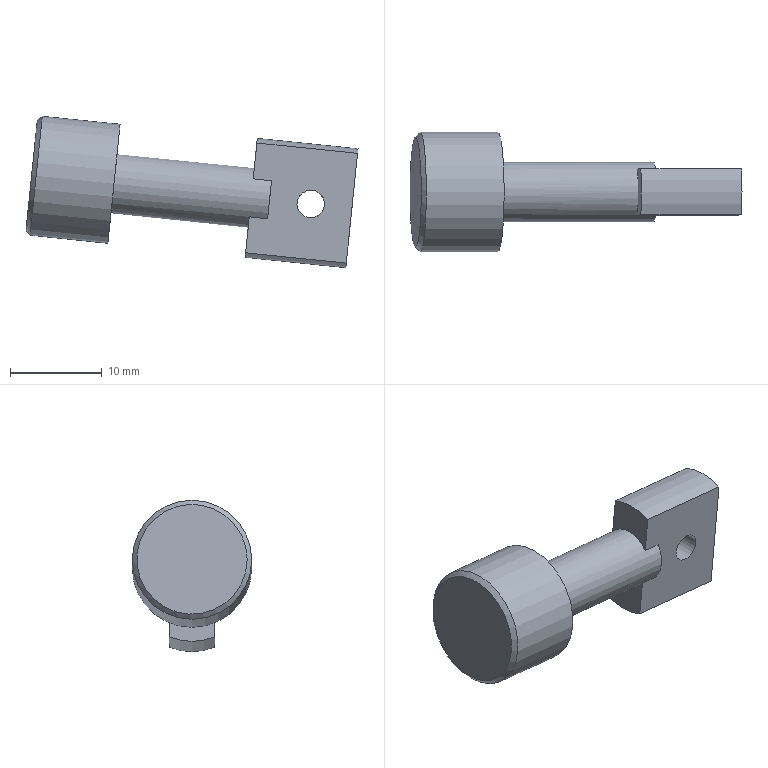Component | NX | PISTON | 1 solid | 15 faces | box 36.09 x 13 x 16.46 mm | volume 2357 mm3 | plane 9 | cylinder 5 | cone 1 | commonest cylinder face diameters 13 x3 6.5 x1 3 x1
STEP:
#1=CARTESIAN_POINT('',(0.,0.,0.));
#2=DIRECTION('',(0.,0.,1.));
#3=DIRECTION('',(1.,0.,0.));
#4=AXIS2_PLACEMENT_3D('',#1,#2,#3);
#5=CARTESIAN_POINT('',(20.798,-27.5,35.026));
#6=VERTEX_POINT('',#5);
#7=CARTESIAN_POINT('',(20.373,-27.5,30.894));
#8=VERTEX_POINT('',#7);
#9=CARTESIAN_POINT('',(20.586,-27.5,32.96));
#10=DIRECTION('',(-0.1022,0.,-0.9948));
#11=VECTOR('',#10,1.);
#12=LINE('',#9,#11);
#13=CARTESIAN_POINT('',(20.586,-30.,32.96));
#14=DIRECTION('',(0.9948,0.,-0.1022));
#15=DIRECTION('',(0.,1.,0.));
#16=AXIS2_PLACEMENT_3D('',#13,#14,#15);
#17=PLANE('',#16);
#18=CARTESIAN_POINT('',(2.5,0.));
#19=DIRECTION('',(0.,-1.));
#20=VECTOR('',#19,1.);
#21=LINE('',#18,#20);
#22=(GEOMETRIC_REPRESENTATION_CONTEXT(2)PARAMETRIC_REPRESENTATION_CONTEXT()REPRESENTATION_CONTEXT('',''));
#23=DEFINITIONAL_REPRESENTATION('',(#21),#22);
#24=PCURVE('',#17,#23);
#25=CARTESIAN_POINT('',(30.152,-27.5,38.009));
#26=DIRECTION('',(0.,1.,0.));
#27=DIRECTION('',(-0.9948,0.,0.1022));
#28=AXIS2_PLACEMENT_3D('',#25,#26,#27);
#29=PLANE('',#28);
#30=CARTESIAN_POINT('',(9.,-6.));
#31=DIRECTION('',(-0.,-1.));
#32=VECTOR('',#31,1.);
#33=LINE('',#30,#32);
#34=(GEOMETRIC_REPRESENTATION_CONTEXT(2)PARAMETRIC_REPRESENTATION_CONTEXT()REPRESENTATION_CONTEXT('',''));
#35=DEFINITIONAL_REPRESENTATION('',(#33),#34);
#36=PCURVE('',#29,#35);
#37=SURFACE_CURVE('',#12,(#24,#36),.PCURVE_S1.);
#38=EDGE_CURVE('',#6,#8,#37,.T.);
#39=ORIENTED_EDGE('',*,*,#38,.T.);
#40=CARTESIAN_POINT('',(20.586,-26.75,32.96));
#41=VERTEX_POINT('',#40);
#42=CARTESIAN_POINT('',(20.586,-30.,32.96));
#43=DIRECTION('',(0.9948,0.,-0.1022));
#44=DIRECTION('',(0.,1.,0.));
#45=AXIS2_PLACEMENT_3D('',#42,#43,#44);
#46=CIRCLE('',#45,3.25);
#47=CARTESIAN_POINT('',(0.,0.));
#48=DIRECTION('',(1.,0.));
#49=AXIS2_PLACEMENT_2D('',#47,#48);
#50=CIRCLE('',#49,3.25);
#51=(GEOMETRIC_REPRESENTATION_CONTEXT(2)PARAMETRIC_REPRESENTATION_CONTEXT()REPRESENTATION_CONTEXT('',''));
#52=DEFINITIONAL_REPRESENTATION('',(#50),#51);
#53=PCURVE('',#17,#52);
#54=CARTESIAN_POINT('',(3.675,-30.,34.698));
#55=DIRECTION('',(0.9948,0.,-0.1022));
#56=DIRECTION('',(0.,1.,0.));
#57=AXIS2_PLACEMENT_3D('',#54,#55,#56);
#58=CYLINDRICAL_SURFACE('',#57,3.25);
#59=CARTESIAN_POINT('',(0.,17.));
#60=DIRECTION('',(1.,0.));
#61=VECTOR('',#60,1.);
#62=LINE('',#59,#61);
#63=(GEOMETRIC_REPRESENTATION_CONTEXT(2)PARAMETRIC_REPRESENTATION_CONTEXT()REPRESENTATION_CONTEXT('',''));
#64=DEFINITIONAL_REPRESENTATION('',(#62),#63);
#65=PCURVE('',#58,#64);
#66=SURFACE_CURVE('',#46,(#53,#65),.PCURVE_S1.);
#67=EDGE_CURVE('',#8,#41,#66,.T.);
#68=ORIENTED_EDGE('',*,*,#67,.T.);
#69=CARTESIAN_POINT('',(20.586,-30.,32.96));
#70=DIRECTION('',(0.9948,0.,-0.1022));
#71=DIRECTION('',(0.,1.,0.));
#72=AXIS2_PLACEMENT_3D('',#69,#70,#71);
#73=CIRCLE('',#72,3.25);
#74=CARTESIAN_POINT('',(0.,0.));
#75=DIRECTION('',(1.,0.));
#76=AXIS2_PLACEMENT_2D('',#74,#75);
#77=CIRCLE('',#76,3.25);
#78=(GEOMETRIC_REPRESENTATION_CONTEXT(2)PARAMETRIC_REPRESENTATION_CONTEXT()REPRESENTATION_CONTEXT('',''));
#79=DEFINITIONAL_REPRESENTATION('',(#77),#78);
#80=PCURVE('',#17,#79);
#81=CARTESIAN_POINT('',(-6.283,17.));
#82=DIRECTION('',(1.,0.));
#83=VECTOR('',#82,1.);
#84=LINE('',#81,#83);
#85=(GEOMETRIC_REPRESENTATION_CONTEXT(2)PARAMETRIC_REPRESENTATION_CONTEXT()REPRESENTATION_CONTEXT('',''));
#86=DEFINITIONAL_REPRESENTATION('',(#84),#85);
#87=PCURVE('',#58,#86);
#88=SURFACE_CURVE('',#73,(#80,#87),.PCURVE_S1.);
#89=EDGE_CURVE('',#41,#6,#88,.T.);
#90=ORIENTED_EDGE('',*,*,#89,.T.);
#91=EDGE_LOOP('',(#39,#68,#90));
#92=FACE_BOUND('',#91,.T.);
#93=ADVANCED_FACE('',(#92),#17,.T.);
#94=CARTESIAN_POINT('',(3.675,-26.75,34.698));
#95=VERTEX_POINT('',#94);
#96=CARTESIAN_POINT('',(3.675,-30.,34.698));
#97=DIRECTION('',(0.9948,0.,-0.1022));
#98=DIRECTION('',(0.,1.,0.));
#99=AXIS2_PLACEMENT_3D('',#96,#97,#98);
#100=CIRCLE('',#99,3.25);
#101=CARTESIAN_POINT('',(3.675,-30.,34.698));
#102=DIRECTION('',(0.9948,0.,-0.1022));
#103=DIRECTION('',(0.,1.,0.));
#104=AXIS2_PLACEMENT_3D('',#101,#102,#103);
#105=PLANE('',#104);
#106=CARTESIAN_POINT('',(0.,0.));
#107=DIRECTION('',(1.,0.));
#108=AXIS2_PLACEMENT_2D('',#106,#107);
#109=CIRCLE('',#108,3.25);
#110=(GEOMETRIC_REPRESENTATION_CONTEXT(2)PARAMETRIC_REPRESENTATION_CONTEXT()REPRESENTATION_CONTEXT('',''));
#111=DEFINITIONAL_REPRESENTATION('',(#109),#110);
#112=PCURVE('',#105,#111);
#113=CARTESIAN_POINT('',(0.,0.));
#114=DIRECTION('',(1.,0.));
#115=VECTOR('',#114,1.);
#116=LINE('',#113,#115);
#117=(GEOMETRIC_REPRESENTATION_CONTEXT(2)PARAMETRIC_REPRESENTATION_CONTEXT()REPRESENTATION_CONTEXT('',''));
#118=DEFINITIONAL_REPRESENTATION('',(#116),#117);
#119=PCURVE('',#58,#118);
#120=SURFACE_CURVE('',#100,(#112,#119),.PCURVE_S1.);
#121=EDGE_CURVE('',#95,#95,#120,.T.);
#122=ORIENTED_EDGE('',*,*,#121,.F.);
#123=EDGE_LOOP('',(#122));
#124=FACE_BOUND('',#123,.T.);
#125=CARTESIAN_POINT('',(3.675,-23.5,34.698));
#126=VERTEX_POINT('',#125);
#127=CARTESIAN_POINT('',(3.675,-30.,34.698));
#128=DIRECTION('',(-0.9948,0.,0.1022));
#129=DIRECTION('',(0.,1.,0.));
#130=AXIS2_PLACEMENT_3D('',#127,#128,#129);
#131=CIRCLE('',#130,6.5);
#132=CARTESIAN_POINT('',(6.5,0.));
#133=CARTESIAN_POINT('',(6.5,-11.258));
#134=CARTESIAN_POINT('',(-3.25,-5.629));
#135=CARTESIAN_POINT('',(-13.,-0.));
#136=CARTESIAN_POINT('',(-3.25,5.629));
#137=CARTESIAN_POINT('',(6.5,11.258));
#138=CARTESIAN_POINT('',(6.5,0.));
#139=(BOUNDED_CURVE()B_SPLINE_CURVE(2,(#132,#133,#134,#135,#136,#137,#138),.UNSPECIFIED.,.T.,.F.)B_SPLINE_CURVE_WITH_KNOTS((1,2,2,2,2,1),(-2.094,0.,2.094,4.189,6.283,8.378),.UNSPECIFIED.)CURVE()GEOMETRIC_REPRESENTATION_ITEM()RATIONAL_B_SPLINE_CURVE((1.,0.5,1.,0.5,1.,0.5,1.))REPRESENTATION_ITEM(''));
#140=(GEOMETRIC_REPRESENTATION_CONTEXT(2)PARAMETRIC_REPRESENTATION_CONTEXT()REPRESENTATION_CONTEXT('',''));
#141=DEFINITIONAL_REPRESENTATION('',(#139),#140);
#142=PCURVE('',#105,#141);
#143=CARTESIAN_POINT('',(-5.278,-30.,35.618));
#144=DIRECTION('',(0.9948,0.,-0.1022));
#145=DIRECTION('',(0.,1.,0.));
#146=AXIS2_PLACEMENT_3D('',#143,#144,#145);
#147=CYLINDRICAL_SURFACE('',#146,6.5);
#148=CARTESIAN_POINT('',(6.283,9.));
#149=DIRECTION('',(-1.,0.));
#150=VECTOR('',#149,1.);
#151=LINE('',#148,#150);
#152=(GEOMETRIC_REPRESENTATION_CONTEXT(2)PARAMETRIC_REPRESENTATION_CONTEXT()REPRESENTATION_CONTEXT('',''));
#153=DEFINITIONAL_REPRESENTATION('',(#151),#152);
#154=PCURVE('',#147,#153);
#155=SURFACE_CURVE('',#131,(#142,#154),.PCURVE_S1.);
#156=EDGE_CURVE('',#126,#126,#155,.T.);
#157=ORIENTED_EDGE('',*,*,#156,.F.);
#158=EDGE_LOOP('',(#157));
#159=FACE_BOUND('',#158,.T.);
#160=ADVANCED_FACE('',(#124,#159),#105,.T.);
#161=CARTESIAN_POINT('',(-5.278,-36.,35.618));
#162=VERTEX_POINT('',#161);
#163=CARTESIAN_POINT('',(-5.278,-30.,35.618));
#164=DIRECTION('',(-0.9948,0.,0.1022));
#165=DIRECTION('',(0.,-1.,0.));
#166=AXIS2_PLACEMENT_3D('',#163,#164,#165);
#167=CIRCLE('',#166,6.);
#168=CARTESIAN_POINT('',(-5.278,-30.,35.618));
#169=DIRECTION('',(-0.9948,0.,0.1022));
#170=DIRECTION('',(0.,-1.,0.));
#171=AXIS2_PLACEMENT_3D('',#168,#169,#170);
#172=PLANE('',#171);
#173=CARTESIAN_POINT('',(0.,0.));
#174=DIRECTION('',(1.,0.));
#175=AXIS2_PLACEMENT_2D('',#173,#174);
#176=CIRCLE('',#175,6.);
#177=(GEOMETRIC_REPRESENTATION_CONTEXT(2)PARAMETRIC_REPRESENTATION_CONTEXT()REPRESENTATION_CONTEXT('',''));
#178=DEFINITIONAL_REPRESENTATION('',(#176),#177);
#179=PCURVE('',#172,#178);
#180=CARTESIAN_POINT('',(-4.781,-30.,35.566));
#181=DIRECTION('',(0.9948,0.,-0.1022));
#182=DIRECTION('',(0.,1.,0.));
#183=AXIS2_PLACEMENT_3D('',#180,#181,#182);
#184=CONICAL_SURFACE('',#183,6.5,0.7854);
#185=CARTESIAN_POINT('',(9.425,-0.5));
#186=DIRECTION('',(-1.,0.));
#187=VECTOR('',#186,1.);
#188=LINE('',#185,#187);
#189=(GEOMETRIC_REPRESENTATION_CONTEXT(2)PARAMETRIC_REPRESENTATION_CONTEXT()REPRESENTATION_CONTEXT('',''));
#190=DEFINITIONAL_REPRESENTATION('',(#188),#189);
#191=PCURVE('',#184,#190);
#192=SURFACE_CURVE('',#167,(#179,#191),.PCURVE_S1.);
#193=EDGE_CURVE('',#162,#162,#192,.T.);
#194=ORIENTED_EDGE('',*,*,#193,.T.);
#195=EDGE_LOOP('',(#194));
#196=FACE_BOUND('',#195,.T.);
#197=ADVANCED_FACE('',(#196),#172,.T.);
#198=CARTESIAN_POINT('',(-4.781,-36.5,35.566));
#199=VERTEX_POINT('',#198);
#200=CARTESIAN_POINT('',(-4.781,-23.5,35.566));
#201=VERTEX_POINT('',#200);
#202=CARTESIAN_POINT('',(-4.781,-30.,35.566));
#203=DIRECTION('',(0.9948,0.,-0.1022));
#204=DIRECTION('',(0.,-1.,0.));
#205=AXIS2_PLACEMENT_3D('',#202,#203,#204);
#206=CIRCLE('',#205,6.5);
#207=CARTESIAN_POINT('',(3.142,0.5));
#208=DIRECTION('',(1.,0.));
#209=VECTOR('',#208,1.);
#210=LINE('',#207,#209);
#211=(GEOMETRIC_REPRESENTATION_CONTEXT(2)PARAMETRIC_REPRESENTATION_CONTEXT()REPRESENTATION_CONTEXT('',''));
#212=DEFINITIONAL_REPRESENTATION('',(#210),#211);
#213=PCURVE('',#147,#212);
#214=CARTESIAN_POINT('',(3.142,0.));
#215=DIRECTION('',(1.,0.));
#216=VECTOR('',#215,1.);
#217=LINE('',#214,#216);
#218=(GEOMETRIC_REPRESENTATION_CONTEXT(2)PARAMETRIC_REPRESENTATION_CONTEXT()REPRESENTATION_CONTEXT('',''));
#219=DEFINITIONAL_REPRESENTATION('',(#217),#218);
#220=PCURVE('',#184,#219);
#221=SURFACE_CURVE('',#206,(#213,#220),.PCURVE_S1.);
#222=EDGE_CURVE('',#199,#201,#221,.T.);
#223=ORIENTED_EDGE('',*,*,#222,.T.);
#224=CARTESIAN_POINT('',(-4.781,-23.5,35.566));
#225=CARTESIAN_POINT('',(3.675,-23.5,34.698));
#226=B_SPLINE_CURVE_WITH_KNOTS('',1,(#224,#225),.UNSPECIFIED.,.F.,.F.,(2,2),(0.5,9.),.PIECEWISE_BEZIER_KNOTS.);
#227=CARTESIAN_POINT('',(6.283,0.));
#228=DIRECTION('',(0.,1.));
#229=VECTOR('',#228,1.);
#230=LINE('',#227,#229);
#231=(GEOMETRIC_REPRESENTATION_CONTEXT(2)PARAMETRIC_REPRESENTATION_CONTEXT()REPRESENTATION_CONTEXT('',''));
#232=DEFINITIONAL_REPRESENTATION('',(#230),#231);
#233=PCURVE('',#147,#232);
#234=CARTESIAN_POINT('',(0.,0.));
#235=DIRECTION('',(0.,1.));
#236=VECTOR('',#235,1.);
#237=LINE('',#234,#236);
#238=(GEOMETRIC_REPRESENTATION_CONTEXT(2)PARAMETRIC_REPRESENTATION_CONTEXT()REPRESENTATION_CONTEXT('',''));
#239=DEFINITIONAL_REPRESENTATION('',(#237),#238);
#240=PCURVE('',#147,#239);
#241=SEAM_CURVE('',#226,(#233,#240),.PCURVE_S1.);
#242=EDGE_CURVE('',#201,#126,#241,.T.);
#243=ORIENTED_EDGE('',*,*,#242,.T.);
#244=ORIENTED_EDGE('',*,*,#156,.T.);
#245=ORIENTED_EDGE('',*,*,#242,.F.);
#246=CARTESIAN_POINT('',(-4.781,-30.,35.566));
#247=DIRECTION('',(0.9948,0.,-0.1022));
#248=DIRECTION('',(0.,-1.,0.));
#249=AXIS2_PLACEMENT_3D('',#246,#247,#248);
#250=CIRCLE('',#249,6.5);
#251=CARTESIAN_POINT('',(-3.142,0.5));
#252=DIRECTION('',(1.,0.));
#253=VECTOR('',#252,1.);
#254=LINE('',#251,#253);
#255=(GEOMETRIC_REPRESENTATION_CONTEXT(2)PARAMETRIC_REPRESENTATION_CONTEXT()REPRESENTATION_CONTEXT('',''));
#256=DEFINITIONAL_REPRESENTATION('',(#254),#255);
#257=PCURVE('',#147,#256);
#258=CARTESIAN_POINT('',(3.142,0.));
#259=DIRECTION('',(1.,0.));
#260=VECTOR('',#259,1.);
#261=LINE('',#258,#260);
#262=(GEOMETRIC_REPRESENTATION_CONTEXT(2)PARAMETRIC_REPRESENTATION_CONTEXT()REPRESENTATION_CONTEXT('',''));
#263=DEFINITIONAL_REPRESENTATION('',(#261),#262);
#264=PCURVE('',#184,#263);
#265=SURFACE_CURVE('',#250,(#257,#264),.PCURVE_S1.);
#266=EDGE_CURVE('',#201,#199,#265,.T.);
#267=ORIENTED_EDGE('',*,*,#266,.T.);
#268=EDGE_LOOP('',(#223,#243,#244,#245,#267));
#269=FACE_BOUND('',#268,.T.);
#270=ADVANCED_FACE('',(#269),#147,.T.);
#271=CARTESIAN_POINT('',(20.373,-32.5,30.894));
#272=VERTEX_POINT('',#271);
#273=CARTESIAN_POINT('',(20.798,-32.5,35.026));
#274=VERTEX_POINT('',#273);
#275=CARTESIAN_POINT('',(20.586,-32.5,32.96));
#276=DIRECTION('',(0.1022,0.,0.9948));
#277=VECTOR('',#276,1.);
#278=LINE('',#275,#277);
#279=CARTESIAN_POINT('',(20.586,-30.,32.96));
#280=DIRECTION('',(0.9948,0.,-0.1022));
#281=DIRECTION('',(0.,1.,0.));
#282=AXIS2_PLACEMENT_3D('',#279,#280,#281);
#283=PLANE('',#282);
#284=CARTESIAN_POINT('',(-2.5,0.));
#285=DIRECTION('',(0.,1.));
#286=VECTOR('',#285,1.);
#287=LINE('',#284,#286);
#288=(GEOMETRIC_REPRESENTATION_CONTEXT(2)PARAMETRIC_REPRESENTATION_CONTEXT()REPRESENTATION_CONTEXT('',''));
#289=DEFINITIONAL_REPRESENTATION('',(#287),#288);
#290=PCURVE('',#283,#289);
#291=CARTESIAN_POINT('',(28.925,-32.5,26.071));
#292=DIRECTION('',(0.,-1.,0.));
#293=DIRECTION('',(0.9948,0.,-0.1022));
#294=AXIS2_PLACEMENT_3D('',#291,#292,#293);
#295=PLANE('',#294);
#296=CARTESIAN_POINT('',(-9.,6.));
#297=DIRECTION('',(-0.,1.));
#298=VECTOR('',#297,1.);
#299=LINE('',#296,#298);
#300=(GEOMETRIC_REPRESENTATION_CONTEXT(2)PARAMETRIC_REPRESENTATION_CONTEXT()REPRESENTATION_CONTEXT('',''));
#301=DEFINITIONAL_REPRESENTATION('',(#299),#300);
#302=PCURVE('',#295,#301);
#303=SURFACE_CURVE('',#278,(#290,#302),.PCURVE_S1.);
#304=EDGE_CURVE('',#272,#274,#303,.T.);
#305=ORIENTED_EDGE('',*,*,#304,.T.);
#306=CARTESIAN_POINT('',(20.586,-30.,32.96));
#307=DIRECTION('',(0.9948,0.,-0.1022));
#308=DIRECTION('',(0.,1.,0.));
#309=AXIS2_PLACEMENT_3D('',#306,#307,#308);
#310=CIRCLE('',#309,3.25);
#311=CARTESIAN_POINT('',(0.,0.));
#312=DIRECTION('',(1.,0.));
#313=AXIS2_PLACEMENT_2D('',#311,#312);
#314=CIRCLE('',#313,3.25);
#315=(GEOMETRIC_REPRESENTATION_CONTEXT(2)PARAMETRIC_REPRESENTATION_CONTEXT()REPRESENTATION_CONTEXT('',''));
#316=DEFINITIONAL_REPRESENTATION('',(#314),#315);
#317=PCURVE('',#283,#316);
#318=CARTESIAN_POINT('',(-0.,17.));
#319=DIRECTION('',(1.,-0.));
#320=VECTOR('',#319,1.);
#321=LINE('',#318,#320);
#322=(GEOMETRIC_REPRESENTATION_CONTEXT(2)PARAMETRIC_REPRESENTATION_CONTEXT()REPRESENTATION_CONTEXT('',''));
#323=DEFINITIONAL_REPRESENTATION('',(#321),#322);
#324=PCURVE('',#58,#323);
#325=SURFACE_CURVE('',#310,(#317,#324),.PCURVE_S1.);
#326=EDGE_CURVE('',#274,#272,#325,.T.);
#327=ORIENTED_EDGE('',*,*,#326,.T.);
#328=EDGE_LOOP('',(#305,#327));
#329=FACE_BOUND('',#328,.T.);
#330=ADVANCED_FACE('',(#329),#283,.T.);
#331=CARTESIAN_POINT('',(18.384,-27.5,31.099));
#332=VERTEX_POINT('',#331);
#333=CARTESIAN_POINT('',(3.463,-27.5,32.632));
#334=DIRECTION('',(0.9948,0.,-0.1022));
#335=VECTOR('',#334,1.);
#336=LINE('',#333,#335);
#337=CARTESIAN_POINT('',(5.59,0.));
#338=DIRECTION('',(0.,1.));
#339=VECTOR('',#338,1.);
#340=LINE('',#337,#339);
#341=(GEOMETRIC_REPRESENTATION_CONTEXT(2)PARAMETRIC_REPRESENTATION_CONTEXT()REPRESENTATION_CONTEXT('',''));
#342=DEFINITIONAL_REPRESENTATION('',(#340),#341);
#343=PCURVE('',#58,#342);
#344=CARTESIAN_POINT('',(26.,-8.077));
#345=DIRECTION('',(-1.,0.));
#346=VECTOR('',#345,1.);
#347=LINE('',#344,#346);
#348=(GEOMETRIC_REPRESENTATION_CONTEXT(2)PARAMETRIC_REPRESENTATION_CONTEXT()REPRESENTATION_CONTEXT('',''));
#349=DEFINITIONAL_REPRESENTATION('',(#347),#348);
#350=PCURVE('',#29,#349);
#351=SURFACE_CURVE('',#336,(#343,#350),.PCURVE_S1.);
#352=EDGE_CURVE('',#332,#8,#351,.T.);
#353=ORIENTED_EDGE('',*,*,#352,.F.);
#354=CARTESIAN_POINT('',(18.384,-32.5,31.099));
#355=VERTEX_POINT('',#354);
#356=CARTESIAN_POINT('',(18.596,-30.,33.164));
#357=DIRECTION('',(0.9948,0.,-0.1022));
#358=DIRECTION('',(0.,-1.,0.));
#359=AXIS2_PLACEMENT_3D('',#356,#357,#358);
#360=CIRCLE('',#359,3.25);
#361=CARTESIAN_POINT('',(3.142,15.));
#362=DIRECTION('',(1.,0.));
#363=VECTOR('',#362,1.);
#364=LINE('',#361,#363);
#365=(GEOMETRIC_REPRESENTATION_CONTEXT(2)PARAMETRIC_REPRESENTATION_CONTEXT()REPRESENTATION_CONTEXT('',''));
#366=DEFINITIONAL_REPRESENTATION('',(#364),#365);
#367=PCURVE('',#58,#366);
#368=CARTESIAN_POINT('',(18.596,-30.,33.164));
#369=DIRECTION('',(-0.9948,0.,0.1022));
#370=DIRECTION('',(0.,-1.,0.));
#371=AXIS2_PLACEMENT_3D('',#368,#369,#370);
#372=PLANE('',#371);
#373=CARTESIAN_POINT('',(3.25,0.));
#374=CARTESIAN_POINT('',(3.25,-5.629));
#375=CARTESIAN_POINT('',(-1.625,-2.815));
#376=CARTESIAN_POINT('',(-6.5,-0.));
#377=CARTESIAN_POINT('',(-1.625,2.815));
#378=CARTESIAN_POINT('',(3.25,5.629));
#379=CARTESIAN_POINT('',(3.25,0.));
#380=(BOUNDED_CURVE()B_SPLINE_CURVE(2,(#373,#374,#375,#376,#377,#378,#379),.UNSPECIFIED.,.T.,.F.)B_SPLINE_CURVE_WITH_KNOTS((1,2,2,2,2,1),(-2.094,0.,2.094,4.189,6.283,8.378),.UNSPECIFIED.)CURVE()GEOMETRIC_REPRESENTATION_ITEM()RATIONAL_B_SPLINE_CURVE((1.,0.5,1.,0.5,1.,0.5,1.))REPRESENTATION_ITEM(''));
#381=(GEOMETRIC_REPRESENTATION_CONTEXT(2)PARAMETRIC_REPRESENTATION_CONTEXT()REPRESENTATION_CONTEXT('',''));
#382=DEFINITIONAL_REPRESENTATION('',(#380),#381);
#383=PCURVE('',#372,#382);
#384=SURFACE_CURVE('',#360,(#367,#383),.PCURVE_S1.);
#385=EDGE_CURVE('',#355,#332,#384,.T.);
#386=ORIENTED_EDGE('',*,*,#385,.F.);
#387=CARTESIAN_POINT('',(3.463,-32.5,32.632));
#388=DIRECTION('',(-0.9948,0.,0.1022));
#389=VECTOR('',#388,1.);
#390=LINE('',#387,#389);
#391=CARTESIAN_POINT('',(3.835,0.));
#392=DIRECTION('',(0.,-1.));
#393=VECTOR('',#392,1.);
#394=LINE('',#391,#393);
#395=(GEOMETRIC_REPRESENTATION_CONTEXT(2)PARAMETRIC_REPRESENTATION_CONTEXT()REPRESENTATION_CONTEXT('',''));
#396=DEFINITIONAL_REPRESENTATION('',(#394),#395);
#397=PCURVE('',#58,#396);
#398=CARTESIAN_POINT('',(-26.,3.923));
#399=DIRECTION('',(-1.,0.));
#400=VECTOR('',#399,1.);
#401=LINE('',#398,#400);
#402=(GEOMETRIC_REPRESENTATION_CONTEXT(2)PARAMETRIC_REPRESENTATION_CONTEXT()REPRESENTATION_CONTEXT('',''));
#403=DEFINITIONAL_REPRESENTATION('',(#401),#402);
#404=PCURVE('',#295,#403);
#405=SURFACE_CURVE('',#390,(#397,#404),.PCURVE_S1.);
#406=EDGE_CURVE('',#272,#355,#405,.T.);
#407=ORIENTED_EDGE('',*,*,#406,.F.);
#408=ORIENTED_EDGE('',*,*,#326,.F.);
#409=CARTESIAN_POINT('',(18.808,-32.5,35.23));
#410=VERTEX_POINT('',#409);
#411=CARTESIAN_POINT('',(3.887,-32.5,36.763));
#412=DIRECTION('',(0.9948,0.,-0.1022));
#413=VECTOR('',#412,1.);
#414=LINE('',#411,#413);
#415=CARTESIAN_POINT('',(2.448,-0.));
#416=DIRECTION('',(0.,1.));
#417=VECTOR('',#416,1.);
#418=LINE('',#415,#417);
#419=(GEOMETRIC_REPRESENTATION_CONTEXT(2)PARAMETRIC_REPRESENTATION_CONTEXT()REPRESENTATION_CONTEXT('',''));
#420=DEFINITIONAL_REPRESENTATION('',(#418),#419);
#421=PCURVE('',#58,#420);
#422=CARTESIAN_POINT('',(-26.,8.077));
#423=DIRECTION('',(1.,-0.));
#424=VECTOR('',#423,1.);
#425=LINE('',#422,#424);
#426=(GEOMETRIC_REPRESENTATION_CONTEXT(2)PARAMETRIC_REPRESENTATION_CONTEXT()REPRESENTATION_CONTEXT('',''));
#427=DEFINITIONAL_REPRESENTATION('',(#425),#426);
#428=PCURVE('',#295,#427);
#429=SURFACE_CURVE('',#414,(#421,#428),.PCURVE_S1.);
#430=EDGE_CURVE('',#410,#274,#429,.T.);
#431=ORIENTED_EDGE('',*,*,#430,.F.);
#432=CARTESIAN_POINT('',(18.808,-27.5,35.23));
#433=VERTEX_POINT('',#432);
#434=CARTESIAN_POINT('',(18.596,-30.,33.164));
#435=DIRECTION('',(0.9948,0.,-0.1022));
#436=DIRECTION('',(0.,-1.,0.));
#437=AXIS2_PLACEMENT_3D('',#434,#435,#436);
#438=CIRCLE('',#437,3.25);
#439=CARTESIAN_POINT('',(-3.142,15.));
#440=DIRECTION('',(1.,0.));
#441=VECTOR('',#440,1.);
#442=LINE('',#439,#441);
#443=(GEOMETRIC_REPRESENTATION_CONTEXT(2)PARAMETRIC_REPRESENTATION_CONTEXT()REPRESENTATION_CONTEXT('',''));
#444=DEFINITIONAL_REPRESENTATION('',(#442),#443);
#445=PCURVE('',#58,#444);
#446=CARTESIAN_POINT('',(18.596,-30.,33.164));
#447=DIRECTION('',(-0.9948,0.,0.1022));
#448=DIRECTION('',(0.,-1.,0.));
#449=AXIS2_PLACEMENT_3D('',#446,#447,#448);
#450=PLANE('',#449);
#451=CARTESIAN_POINT('',(3.25,0.));
#452=CARTESIAN_POINT('',(3.25,-5.629));
#453=CARTESIAN_POINT('',(-1.625,-2.815));
#454=CARTESIAN_POINT('',(-6.5,-0.));
#455=CARTESIAN_POINT('',(-1.625,2.815));
#456=CARTESIAN_POINT('',(3.25,5.629));
#457=CARTESIAN_POINT('',(3.25,0.));
#458=(BOUNDED_CURVE()B_SPLINE_CURVE(2,(#451,#452,#453,#454,#455,#456,#457),.UNSPECIFIED.,.T.,.F.)B_SPLINE_CURVE_WITH_KNOTS((1,2,2,2,2,1),(-2.094,0.,2.094,4.189,6.283,8.378),.UNSPECIFIED.)CURVE()GEOMETRIC_REPRESENTATION_ITEM()RATIONAL_B_SPLINE_CURVE((1.,0.5,1.,0.5,1.,0.5,1.))REPRESENTATION_ITEM(''));
#459=(GEOMETRIC_REPRESENTATION_CONTEXT(2)PARAMETRIC_REPRESENTATION_CONTEXT()REPRESENTATION_CONTEXT('',''));
#460=DEFINITIONAL_REPRESENTATION('',(#458),#459);
#461=PCURVE('',#450,#460);
#462=SURFACE_CURVE('',#438,(#445,#461),.PCURVE_S1.);
#463=EDGE_CURVE('',#433,#410,#462,.T.);
#464=ORIENTED_EDGE('',*,*,#463,.F.);
#465=CARTESIAN_POINT('',(3.887,-27.5,36.763));
#466=DIRECTION('',(-0.9948,0.,0.1022));
#467=VECTOR('',#466,1.);
#468=LINE('',#465,#467);
#469=CARTESIAN_POINT('',(0.6932,-0.));
#470=DIRECTION('',(0.,-1.));
#471=VECTOR('',#470,1.);
#472=LINE('',#469,#471);
#473=(GEOMETRIC_REPRESENTATION_CONTEXT(2)PARAMETRIC_REPRESENTATION_CONTEXT()REPRESENTATION_CONTEXT('',''));
#474=DEFINITIONAL_REPRESENTATION('',(#472),#473);
#475=PCURVE('',#58,#474);
#476=CARTESIAN_POINT('',(26.,-3.923));
#477=DIRECTION('',(1.,0.));
#478=VECTOR('',#477,1.);
#479=LINE('',#476,#478);
#480=(GEOMETRIC_REPRESENTATION_CONTEXT(2)PARAMETRIC_REPRESENTATION_CONTEXT()REPRESENTATION_CONTEXT('',''));
#481=DEFINITIONAL_REPRESENTATION('',(#479),#480);
#482=PCURVE('',#29,#481);
#483=SURFACE_CURVE('',#468,(#475,#482),.PCURVE_S1.);
#484=EDGE_CURVE('',#6,#433,#483,.T.);
#485=ORIENTED_EDGE('',*,*,#484,.F.);
#486=ORIENTED_EDGE('',*,*,#89,.F.);
#487=CARTESIAN_POINT('',(3.675,-26.75,34.698));
#488=CARTESIAN_POINT('',(20.586,-26.75,32.96));
#489=B_SPLINE_CURVE_WITH_KNOTS('',1,(#487,#488),.UNSPECIFIED.,.F.,.F.,(2,2),(0.,17.),.PIECEWISE_BEZIER_KNOTS.);
#490=CARTESIAN_POINT('',(0.,0.));
#491=DIRECTION('',(0.,1.));
#492=VECTOR('',#491,1.);
#493=LINE('',#490,#492);
#494=(GEOMETRIC_REPRESENTATION_CONTEXT(2)PARAMETRIC_REPRESENTATION_CONTEXT()REPRESENTATION_CONTEXT('',''));
#495=DEFINITIONAL_REPRESENTATION('',(#493),#494);
#496=PCURVE('',#58,#495);
#497=CARTESIAN_POINT('',(6.283,0.));
#498=DIRECTION('',(0.,1.));
#499=VECTOR('',#498,1.);
#500=LINE('',#497,#499);
#501=(GEOMETRIC_REPRESENTATION_CONTEXT(2)PARAMETRIC_REPRESENTATION_CONTEXT()REPRESENTATION_CONTEXT('',''));
#502=DEFINITIONAL_REPRESENTATION('',(#500),#501);
#503=PCURVE('',#58,#502);
#504=SEAM_CURVE('',#489,(#496,#503),.PCURVE_S1.);
#505=EDGE_CURVE('',#95,#41,#504,.T.);
#506=ORIENTED_EDGE('',*,*,#505,.F.);
#507=ORIENTED_EDGE('',*,*,#121,.T.);
#508=ORIENTED_EDGE('',*,*,#505,.T.);
#509=ORIENTED_EDGE('',*,*,#67,.F.);
#510=EDGE_LOOP('',(#353,#386,#407,#408,#431,#464,#485,#486,#506,#507,#508,#509));
#511=FACE_BOUND('',#510,.T.);
#512=ADVANCED_FACE('',(#511),#58,.T.);
#513=CARTESIAN_POINT('',(17.983,-32.5,27.196));
#514=VERTEX_POINT('',#513);
#515=CARTESIAN_POINT('',(17.983,-32.5,27.196));
#516=DIRECTION('',(0.1022,0.,0.9948));
#517=VECTOR('',#516,1.);
#518=LINE('',#515,#517);
#519=CARTESIAN_POINT('',(2.5,-6.));
#520=DIRECTION('',(0.,1.));
#521=VECTOR('',#520,1.);
#522=LINE('',#519,#521);
#523=(GEOMETRIC_REPRESENTATION_CONTEXT(2)PARAMETRIC_REPRESENTATION_CONTEXT()REPRESENTATION_CONTEXT('',''));
#524=DEFINITIONAL_REPRESENTATION('',(#522),#523);
#525=PCURVE('',#372,#524);
#526=CARTESIAN_POINT('',(-11.,-0.));
#527=DIRECTION('',(-0.,1.));
#528=VECTOR('',#527,1.);
#529=LINE('',#526,#528);
#530=(GEOMETRIC_REPRESENTATION_CONTEXT(2)PARAMETRIC_REPRESENTATION_CONTEXT()REPRESENTATION_CONTEXT('',''));
#531=DEFINITIONAL_REPRESENTATION('',(#529),#530);
#532=PCURVE('',#295,#531);
#533=SURFACE_CURVE('',#518,(#525,#532),.PCURVE_S1.);
#534=EDGE_CURVE('',#514,#355,#533,.T.);
#535=ORIENTED_EDGE('',*,*,#534,.T.);
#536=ORIENTED_EDGE('',*,*,#385,.T.);
#537=CARTESIAN_POINT('',(17.983,-27.5,27.196));
#538=VERTEX_POINT('',#537);
#539=CARTESIAN_POINT('',(19.21,-27.5,39.133));
#540=DIRECTION('',(-0.1022,0.,-0.9948));
#541=VECTOR('',#540,1.);
#542=LINE('',#539,#541);
#543=CARTESIAN_POINT('',(-2.5,6.));
#544=DIRECTION('',(0.,-1.));
#545=VECTOR('',#544,1.);
#546=LINE('',#543,#545);
#547=(GEOMETRIC_REPRESENTATION_CONTEXT(2)PARAMETRIC_REPRESENTATION_CONTEXT()REPRESENTATION_CONTEXT('',''));
#548=DEFINITIONAL_REPRESENTATION('',(#546),#547);
#549=PCURVE('',#372,#548);
#550=CARTESIAN_POINT('',(11.,-0.));
#551=DIRECTION('',(-0.,-1.));
#552=VECTOR('',#551,1.);
#553=LINE('',#550,#552);
#554=(GEOMETRIC_REPRESENTATION_CONTEXT(2)PARAMETRIC_REPRESENTATION_CONTEXT()REPRESENTATION_CONTEXT('',''));
#555=DEFINITIONAL_REPRESENTATION('',(#553),#554);
#556=PCURVE('',#29,#555);
#557=SURFACE_CURVE('',#542,(#549,#556),.PCURVE_S1.);
#558=EDGE_CURVE('',#332,#538,#557,.T.);
#559=ORIENTED_EDGE('',*,*,#558,.T.);
#560=CARTESIAN_POINT('',(18.596,-30.,33.164));
#561=DIRECTION('',(-0.9948,0.,0.1022));
#562=DIRECTION('',(0.,1.,0.));
#563=AXIS2_PLACEMENT_3D('',#560,#561,#562);
#564=CIRCLE('',#563,6.5);
#565=CARTESIAN_POINT('',(0.,0.));
#566=DIRECTION('',(-1.,0.));
#567=AXIS2_PLACEMENT_2D('',#565,#566);
#568=CIRCLE('',#567,6.5);
#569=(GEOMETRIC_REPRESENTATION_CONTEXT(2)PARAMETRIC_REPRESENTATION_CONTEXT()REPRESENTATION_CONTEXT('',''));
#570=DEFINITIONAL_REPRESENTATION('',(#568),#569);
#571=PCURVE('',#372,#570);
#572=CARTESIAN_POINT('',(29.539,-30.,32.04));
#573=DIRECTION('',(-0.9948,0.,0.1022));
#574=DIRECTION('',(0.,-1.,0.));
#575=AXIS2_PLACEMENT_3D('',#572,#573,#574);
#576=CYLINDRICAL_SURFACE('',#575,6.5);
#577=CARTESIAN_POINT('',(3.142,11.));
#578=DIRECTION('',(1.,-0.));
#579=VECTOR('',#578,1.);
#580=LINE('',#577,#579);
#581=(GEOMETRIC_REPRESENTATION_CONTEXT(2)PARAMETRIC_REPRESENTATION_CONTEXT()REPRESENTATION_CONTEXT('',''));
#582=DEFINITIONAL_REPRESENTATION('',(#580),#581);
#583=PCURVE('',#576,#582);
#584=SURFACE_CURVE('',#564,(#571,#583),.PCURVE_S1.);
#585=EDGE_CURVE('',#538,#514,#584,.T.);
#586=ORIENTED_EDGE('',*,*,#585,.T.);
#587=EDGE_LOOP('',(#535,#536,#559,#586));
#588=FACE_BOUND('',#587,.T.);
#589=ADVANCED_FACE('',(#588),#372,.T.);
#590=CARTESIAN_POINT('',(25.216,-27.5,33.992));
#591=VERTEX_POINT('',#590);
#592=CARTESIAN_POINT('',(25.062,-27.5,32.5));
#593=DIRECTION('',(0.,-1.,0.));
#594=DIRECTION('',(0.1022,0.,0.9948));
#595=AXIS2_PLACEMENT_3D('',#592,#593,#594);
#596=CIRCLE('',#595,1.5);
#597=CARTESIAN_POINT('',(4.5,-4.5));
#598=CARTESIAN_POINT('',(7.098,-4.5));
#599=CARTESIAN_POINT('',(5.799,-6.75));
#600=CARTESIAN_POINT('',(4.5,-9.));
#601=CARTESIAN_POINT('',(3.201,-6.75));
#602=CARTESIAN_POINT('',(1.902,-4.5));
#603=CARTESIAN_POINT('',(4.5,-4.5));
#604=(BOUNDED_CURVE()B_SPLINE_CURVE(2,(#597,#598,#599,#600,#601,#602,#603),.UNSPECIFIED.,.T.,.F.)B_SPLINE_CURVE_WITH_KNOTS((1,2,2,2,2,1),(-2.094,0.,2.094,4.189,6.283,8.378),.UNSPECIFIED.)CURVE()GEOMETRIC_REPRESENTATION_ITEM()RATIONAL_B_SPLINE_CURVE((1.,0.5,1.,0.5,1.,0.5,1.))REPRESENTATION_ITEM(''));
#605=(GEOMETRIC_REPRESENTATION_CONTEXT(2)PARAMETRIC_REPRESENTATION_CONTEXT()REPRESENTATION_CONTEXT('',''));
#606=DEFINITIONAL_REPRESENTATION('',(#604),#605);
#607=PCURVE('',#29,#606);
#608=CARTESIAN_POINT('',(25.062,-37.5,32.5));
#609=DIRECTION('',(0.,1.,0.));
#610=DIRECTION('',(-0.9948,0.,0.1022));
#611=AXIS2_PLACEMENT_3D('',#608,#609,#610);
#612=CYLINDRICAL_SURFACE('',#611,1.5);
#613=CARTESIAN_POINT('',(7.854,10.));
#614=DIRECTION('',(-1.,0.));
#615=VECTOR('',#614,1.);
#616=LINE('',#613,#615);
#617=(GEOMETRIC_REPRESENTATION_CONTEXT(2)PARAMETRIC_REPRESENTATION_CONTEXT()REPRESENTATION_CONTEXT('',''));
#618=DEFINITIONAL_REPRESENTATION('',(#616),#617);
#619=PCURVE('',#612,#618);
#620=SURFACE_CURVE('',#596,(#607,#619),.PCURVE_S1.);
#621=EDGE_CURVE('',#591,#591,#620,.T.);
#622=ORIENTED_EDGE('',*,*,#621,.T.);
#623=EDGE_LOOP('',(#622));
#624=FACE_BOUND('',#623,.T.);
#625=ORIENTED_EDGE('',*,*,#38,.F.);
#626=ORIENTED_EDGE('',*,*,#484,.T.);
#627=CARTESIAN_POINT('',(19.21,-27.5,39.133));
#628=VERTEX_POINT('',#627);
#629=CARTESIAN_POINT('',(19.21,-27.5,39.133));
#630=DIRECTION('',(-0.1022,0.,-0.9948));
#631=VECTOR('',#630,1.);
#632=LINE('',#629,#631);
#633=CARTESIAN_POINT('',(11.,-0.));
#634=DIRECTION('',(-0.,-1.));
#635=VECTOR('',#634,1.);
#636=LINE('',#633,#635);
#637=(GEOMETRIC_REPRESENTATION_CONTEXT(2)PARAMETRIC_REPRESENTATION_CONTEXT()REPRESENTATION_CONTEXT('',''));
#638=DEFINITIONAL_REPRESENTATION('',(#636),#637);
#639=PCURVE('',#29,#638);
#640=CARTESIAN_POINT('',(-2.5,6.));
#641=DIRECTION('',(0.,-1.));
#642=VECTOR('',#641,1.);
#643=LINE('',#640,#642);
#644=(GEOMETRIC_REPRESENTATION_CONTEXT(2)PARAMETRIC_REPRESENTATION_CONTEXT()REPRESENTATION_CONTEXT('',''));
#645=DEFINITIONAL_REPRESENTATION('',(#643),#644);
#646=PCURVE('',#450,#645);
#647=SURFACE_CURVE('',#632,(#639,#646),.PCURVE_S1.);
#648=EDGE_CURVE('',#628,#433,#647,.T.);
#649=ORIENTED_EDGE('',*,*,#648,.F.);
#650=CARTESIAN_POINT('',(30.152,-27.5,38.009));
#651=VERTEX_POINT('',#650);
#652=CARTESIAN_POINT('',(30.152,-27.5,38.009));
#653=DIRECTION('',(-0.9948,0.,0.1022));
#654=VECTOR('',#653,1.);
#655=LINE('',#652,#654);
#656=CARTESIAN_POINT('',(0.,0.));
#657=DIRECTION('',(1.,0.));
#658=VECTOR('',#657,1.);
#659=LINE('',#656,#658);
#660=(GEOMETRIC_REPRESENTATION_CONTEXT(2)PARAMETRIC_REPRESENTATION_CONTEXT()REPRESENTATION_CONTEXT('',''));
#661=DEFINITIONAL_REPRESENTATION('',(#659),#660);
#662=PCURVE('',#29,#661);
#663=CARTESIAN_POINT('',(29.539,-30.,32.04));
#664=DIRECTION('',(-0.9948,0.,0.1022));
#665=DIRECTION('',(0.,-1.,0.));
#666=AXIS2_PLACEMENT_3D('',#663,#664,#665);
#667=CYLINDRICAL_SURFACE('',#666,6.5);
#668=CARTESIAN_POINT('',(1.966,-0.));
#669=DIRECTION('',(0.,1.));
#670=VECTOR('',#669,1.);
#671=LINE('',#668,#670);
#672=(GEOMETRIC_REPRESENTATION_CONTEXT(2)PARAMETRIC_REPRESENTATION_CONTEXT()REPRESENTATION_CONTEXT('',''));
#673=DEFINITIONAL_REPRESENTATION('',(#671),#672);
#674=PCURVE('',#667,#673);
#675=SURFACE_CURVE('',#655,(#662,#674),.PCURVE_S1.);
#676=EDGE_CURVE('',#651,#628,#675,.T.);
#677=ORIENTED_EDGE('',*,*,#676,.F.);
#678=CARTESIAN_POINT('',(28.925,-27.5,26.071));
#679=VERTEX_POINT('',#678);
#680=CARTESIAN_POINT('',(30.152,-27.5,38.009));
#681=DIRECTION('',(-0.1022,0.,-0.9948));
#682=VECTOR('',#681,1.);
#683=LINE('',#680,#682);
#684=CARTESIAN_POINT('',(0.,0.));
#685=DIRECTION('',(-0.,-1.));
#686=VECTOR('',#685,1.);
#687=LINE('',#684,#686);
#688=(GEOMETRIC_REPRESENTATION_CONTEXT(2)PARAMETRIC_REPRESENTATION_CONTEXT()REPRESENTATION_CONTEXT('',''));
#689=DEFINITIONAL_REPRESENTATION('',(#687),#688);
#690=PCURVE('',#29,#689);
#691=CARTESIAN_POINT('',(29.539,-30.,32.04));
#692=DIRECTION('',(-0.9948,0.,0.1022));
#693=DIRECTION('',(0.,-1.,0.));
#694=AXIS2_PLACEMENT_3D('',#691,#692,#693);
#695=PLANE('',#694);
#696=CARTESIAN_POINT('',(-2.5,6.));
#697=DIRECTION('',(0.,-1.));
#698=VECTOR('',#697,1.);
#699=LINE('',#696,#698);
#700=(GEOMETRIC_REPRESENTATION_CONTEXT(2)PARAMETRIC_REPRESENTATION_CONTEXT()REPRESENTATION_CONTEXT('',''));
#701=DEFINITIONAL_REPRESENTATION('',(#699),#700);
#702=PCURVE('',#695,#701);
#703=SURFACE_CURVE('',#683,(#690,#702),.PCURVE_S1.);
#704=EDGE_CURVE('',#651,#679,#703,.T.);
#705=ORIENTED_EDGE('',*,*,#704,.T.);
#706=CARTESIAN_POINT('',(28.925,-27.5,26.071));
#707=DIRECTION('',(-0.9948,0.,0.1022));
#708=VECTOR('',#707,1.);
#709=LINE('',#706,#708);
#710=CARTESIAN_POINT('',(0.,-12.));
#711=DIRECTION('',(1.,0.));
#712=VECTOR('',#711,1.);
#713=LINE('',#710,#712);
#714=(GEOMETRIC_REPRESENTATION_CONTEXT(2)PARAMETRIC_REPRESENTATION_CONTEXT()REPRESENTATION_CONTEXT('',''));
#715=DEFINITIONAL_REPRESENTATION('',(#713),#714);
#716=PCURVE('',#29,#715);
#717=CARTESIAN_POINT('',(4.318,-0.));
#718=DIRECTION('',(0.,1.));
#719=VECTOR('',#718,1.);
#720=LINE('',#717,#719);
#721=(GEOMETRIC_REPRESENTATION_CONTEXT(2)PARAMETRIC_REPRESENTATION_CONTEXT()REPRESENTATION_CONTEXT('',''));
#722=DEFINITIONAL_REPRESENTATION('',(#720),#721);
#723=PCURVE('',#576,#722);
#724=SURFACE_CURVE('',#709,(#716,#723),.PCURVE_S1.);
#725=EDGE_CURVE('',#679,#538,#724,.T.);
#726=ORIENTED_EDGE('',*,*,#725,.T.);
#727=ORIENTED_EDGE('',*,*,#558,.F.);
#728=ORIENTED_EDGE('',*,*,#352,.T.);
#729=EDGE_LOOP('',(#625,#626,#649,#677,#705,#726,#727,#728));
#730=FACE_BOUND('',#729,.T.);
#731=ADVANCED_FACE('',(#624,#730),#29,.T.);
#732=ORIENTED_EDGE('',*,*,#585,.F.);
#733=ORIENTED_EDGE('',*,*,#725,.F.);
#734=CARTESIAN_POINT('',(28.925,-32.5,26.071));
#735=VERTEX_POINT('',#734);
#736=CARTESIAN_POINT('',(29.539,-30.,32.04));
#737=DIRECTION('',(-0.9948,0.,0.1022));
#738=DIRECTION('',(0.,1.,0.));
#739=AXIS2_PLACEMENT_3D('',#736,#737,#738);
#740=CIRCLE('',#739,6.5);
#741=CARTESIAN_POINT('',(3.142,-0.));
#742=DIRECTION('',(1.,0.));
#743=VECTOR('',#742,1.);
#744=LINE('',#741,#743);
#745=(GEOMETRIC_REPRESENTATION_CONTEXT(2)PARAMETRIC_REPRESENTATION_CONTEXT()REPRESENTATION_CONTEXT('',''));
#746=DEFINITIONAL_REPRESENTATION('',(#744),#745);
#747=PCURVE('',#576,#746);
#748=CARTESIAN_POINT('',(0.,0.));
#749=DIRECTION('',(-1.,0.));
#750=AXIS2_PLACEMENT_2D('',#748,#749);
#751=CIRCLE('',#750,6.5);
#752=(GEOMETRIC_REPRESENTATION_CONTEXT(2)PARAMETRIC_REPRESENTATION_CONTEXT()REPRESENTATION_CONTEXT('',''));
#753=DEFINITIONAL_REPRESENTATION('',(#751),#752);
#754=PCURVE('',#695,#753);
#755=SURFACE_CURVE('',#740,(#747,#754),.PCURVE_S1.);
#756=EDGE_CURVE('',#679,#735,#755,.T.);
#757=ORIENTED_EDGE('',*,*,#756,.T.);
#758=CARTESIAN_POINT('',(28.925,-32.5,26.071));
#759=DIRECTION('',(-0.9948,0.,0.1022));
#760=VECTOR('',#759,1.);
#761=LINE('',#758,#760);
#762=CARTESIAN_POINT('',(5.107,-0.));
#763=DIRECTION('',(0.,1.));
#764=VECTOR('',#763,1.);
#765=LINE('',#762,#764);
#766=(GEOMETRIC_REPRESENTATION_CONTEXT(2)PARAMETRIC_REPRESENTATION_CONTEXT()REPRESENTATION_CONTEXT('',''));
#767=DEFINITIONAL_REPRESENTATION('',(#765),#766);
#768=PCURVE('',#576,#767);
#769=CARTESIAN_POINT('',(0.,0.));
#770=DIRECTION('',(-1.,0.));
#771=VECTOR('',#770,1.);
#772=LINE('',#769,#771);
#773=(GEOMETRIC_REPRESENTATION_CONTEXT(2)PARAMETRIC_REPRESENTATION_CONTEXT()REPRESENTATION_CONTEXT('',''));
#774=DEFINITIONAL_REPRESENTATION('',(#772),#773);
#775=PCURVE('',#295,#774);
#776=SURFACE_CURVE('',#761,(#768,#775),.PCURVE_S1.);
#777=EDGE_CURVE('',#735,#514,#776,.T.);
#778=ORIENTED_EDGE('',*,*,#777,.T.);
#779=EDGE_LOOP('',(#732,#733,#757,#778));
#780=FACE_BOUND('',#779,.T.);
#781=ADVANCED_FACE('',(#780),#576,.T.);
#782=CARTESIAN_POINT('',(26.554,-32.5,32.347));
#783=VERTEX_POINT('',#782);
#784=CARTESIAN_POINT('',(25.216,-32.5,33.992));
#785=VERTEX_POINT('',#784);
#786=CARTESIAN_POINT('',(25.062,-32.5,32.5));
#787=DIRECTION('',(0.,1.,0.));
#788=DIRECTION('',(0.9948,0.,-0.1022));
#789=AXIS2_PLACEMENT_3D('',#786,#787,#788);
#790=CIRCLE('',#789,1.5);
#791=CARTESIAN_POINT('',(-3.,6.));
#792=CARTESIAN_POINT('',(-3.,3.402));
#793=CARTESIAN_POINT('',(-5.25,4.701));
#794=CARTESIAN_POINT('',(-7.5,6.));
#795=CARTESIAN_POINT('',(-5.25,7.299));
#796=CARTESIAN_POINT('',(-3.,8.598));
#797=CARTESIAN_POINT('',(-3.,6.));
#798=(BOUNDED_CURVE()B_SPLINE_CURVE(2,(#791,#792,#793,#794,#795,#796,#797),.UNSPECIFIED.,.T.,.F.)B_SPLINE_CURVE_WITH_KNOTS((1,2,2,2,2,1),(-2.094,0.,2.094,4.189,6.283,8.378),.UNSPECIFIED.)CURVE()GEOMETRIC_REPRESENTATION_ITEM()RATIONAL_B_SPLINE_CURVE((1.,0.5,1.,0.5,1.,0.5,1.))REPRESENTATION_ITEM(''));
#799=(GEOMETRIC_REPRESENTATION_CONTEXT(2)PARAMETRIC_REPRESENTATION_CONTEXT()REPRESENTATION_CONTEXT('',''));
#800=DEFINITIONAL_REPRESENTATION('',(#798),#799);
#801=PCURVE('',#295,#800);
#802=CARTESIAN_POINT('',(3.142,5.));
#803=DIRECTION('',(1.,0.));
#804=VECTOR('',#803,1.);
#805=LINE('',#802,#804);
#806=(GEOMETRIC_REPRESENTATION_CONTEXT(2)PARAMETRIC_REPRESENTATION_CONTEXT()REPRESENTATION_CONTEXT('',''));
#807=DEFINITIONAL_REPRESENTATION('',(#805),#806);
#808=PCURVE('',#612,#807);
#809=SURFACE_CURVE('',#790,(#801,#808),.PCURVE_S1.);
#810=EDGE_CURVE('',#783,#785,#809,.T.);
#811=ORIENTED_EDGE('',*,*,#810,.T.);
#812=CARTESIAN_POINT('',(25.062,-32.5,32.5));
#813=DIRECTION('',(0.,1.,0.));
#814=DIRECTION('',(0.9948,0.,-0.1022));
#815=AXIS2_PLACEMENT_3D('',#812,#813,#814);
#816=CIRCLE('',#815,1.5);
#817=CARTESIAN_POINT('',(-3.,6.));
#818=CARTESIAN_POINT('',(-3.,3.402));
#819=CARTESIAN_POINT('',(-5.25,4.701));
#820=CARTESIAN_POINT('',(-7.5,6.));
#821=CARTESIAN_POINT('',(-5.25,7.299));
#822=CARTESIAN_POINT('',(-3.,8.598));
#823=CARTESIAN_POINT('',(-3.,6.));
#824=(BOUNDED_CURVE()B_SPLINE_CURVE(2,(#817,#818,#819,#820,#821,#822,#823),.UNSPECIFIED.,.T.,.F.)B_SPLINE_CURVE_WITH_KNOTS((1,2,2,2,2,1),(-2.094,0.,2.094,4.189,6.283,8.378),.UNSPECIFIED.)CURVE()GEOMETRIC_REPRESENTATION_ITEM()RATIONAL_B_SPLINE_CURVE((1.,0.5,1.,0.5,1.,0.5,1.))REPRESENTATION_ITEM(''));
#825=(GEOMETRIC_REPRESENTATION_CONTEXT(2)PARAMETRIC_REPRESENTATION_CONTEXT()REPRESENTATION_CONTEXT('',''));
#826=DEFINITIONAL_REPRESENTATION('',(#824),#825);
#827=PCURVE('',#295,#826);
#828=CARTESIAN_POINT('',(-3.142,5.));
#829=DIRECTION('',(1.,0.));
#830=VECTOR('',#829,1.);
#831=LINE('',#828,#830);
#832=(GEOMETRIC_REPRESENTATION_CONTEXT(2)PARAMETRIC_REPRESENTATION_CONTEXT()REPRESENTATION_CONTEXT('',''));
#833=DEFINITIONAL_REPRESENTATION('',(#831),#832);
#834=PCURVE('',#612,#833);
#835=SURFACE_CURVE('',#816,(#827,#834),.PCURVE_S1.);
#836=EDGE_CURVE('',#785,#783,#835,.T.);
#837=ORIENTED_EDGE('',*,*,#836,.T.);
#838=EDGE_LOOP('',(#811,#837));
#839=FACE_BOUND('',#838,.T.);
#840=ORIENTED_EDGE('',*,*,#304,.F.);
#841=ORIENTED_EDGE('',*,*,#406,.T.);
#842=ORIENTED_EDGE('',*,*,#534,.F.);
#843=ORIENTED_EDGE('',*,*,#777,.F.);
#844=CARTESIAN_POINT('',(30.152,-32.5,38.009));
#845=VERTEX_POINT('',#844);
#846=CARTESIAN_POINT('',(28.925,-32.5,26.071));
#847=DIRECTION('',(0.1022,0.,0.9948));
#848=VECTOR('',#847,1.);
#849=LINE('',#846,#848);
#850=CARTESIAN_POINT('',(0.,0.));
#851=DIRECTION('',(-0.,1.));
#852=VECTOR('',#851,1.);
#853=LINE('',#850,#852);
#854=(GEOMETRIC_REPRESENTATION_CONTEXT(2)PARAMETRIC_REPRESENTATION_CONTEXT()REPRESENTATION_CONTEXT('',''));
#855=DEFINITIONAL_REPRESENTATION('',(#853),#854);
#856=PCURVE('',#295,#855);
#857=CARTESIAN_POINT('',(2.5,-6.));
#858=DIRECTION('',(0.,1.));
#859=VECTOR('',#858,1.);
#860=LINE('',#857,#859);
#861=(GEOMETRIC_REPRESENTATION_CONTEXT(2)PARAMETRIC_REPRESENTATION_CONTEXT()REPRESENTATION_CONTEXT('',''));
#862=DEFINITIONAL_REPRESENTATION('',(#860),#861);
#863=PCURVE('',#695,#862);
#864=SURFACE_CURVE('',#849,(#856,#863),.PCURVE_S1.);
#865=EDGE_CURVE('',#735,#845,#864,.T.);
#866=ORIENTED_EDGE('',*,*,#865,.T.);
#867=CARTESIAN_POINT('',(19.21,-32.5,39.133));
#868=VERTEX_POINT('',#867);
#869=CARTESIAN_POINT('',(30.152,-32.5,38.009));
#870=DIRECTION('',(-0.9948,0.,0.1022));
#871=VECTOR('',#870,1.);
#872=LINE('',#869,#871);
#873=CARTESIAN_POINT('',(0.,12.));
#874=DIRECTION('',(-1.,0.));
#875=VECTOR('',#874,1.);
#876=LINE('',#873,#875);
#877=(GEOMETRIC_REPRESENTATION_CONTEXT(2)PARAMETRIC_REPRESENTATION_CONTEXT()REPRESENTATION_CONTEXT('',''));
#878=DEFINITIONAL_REPRESENTATION('',(#876),#877);
#879=PCURVE('',#295,#878);
#880=CARTESIAN_POINT('',(1.176,-0.));
#881=DIRECTION('',(0.,1.));
#882=VECTOR('',#881,1.);
#883=LINE('',#880,#882);
#884=(GEOMETRIC_REPRESENTATION_CONTEXT(2)PARAMETRIC_REPRESENTATION_CONTEXT()REPRESENTATION_CONTEXT('',''));
#885=DEFINITIONAL_REPRESENTATION('',(#883),#884);
#886=PCURVE('',#667,#885);
#887=SURFACE_CURVE('',#872,(#879,#886),.PCURVE_S1.);
#888=EDGE_CURVE('',#845,#868,#887,.T.);
#889=ORIENTED_EDGE('',*,*,#888,.T.);
#890=CARTESIAN_POINT('',(17.983,-32.5,27.196));
#891=DIRECTION('',(0.1022,0.,0.9948));
#892=VECTOR('',#891,1.);
#893=LINE('',#890,#892);
#894=CARTESIAN_POINT('',(-11.,-0.));
#895=DIRECTION('',(-0.,1.));
#896=VECTOR('',#895,1.);
#897=LINE('',#894,#896);
#898=(GEOMETRIC_REPRESENTATION_CONTEXT(2)PARAMETRIC_REPRESENTATION_CONTEXT()REPRESENTATION_CONTEXT('',''));
#899=DEFINITIONAL_REPRESENTATION('',(#897),#898);
#900=PCURVE('',#295,#899);
#901=CARTESIAN_POINT('',(2.5,-6.));
#902=DIRECTION('',(0.,1.));
#903=VECTOR('',#902,1.);
#904=LINE('',#901,#903);
#905=(GEOMETRIC_REPRESENTATION_CONTEXT(2)PARAMETRIC_REPRESENTATION_CONTEXT()REPRESENTATION_CONTEXT('',''));
#906=DEFINITIONAL_REPRESENTATION('',(#904),#905);
#907=PCURVE('',#450,#906);
#908=SURFACE_CURVE('',#893,(#900,#907),.PCURVE_S1.);
#909=EDGE_CURVE('',#410,#868,#908,.T.);
#910=ORIENTED_EDGE('',*,*,#909,.F.);
#911=ORIENTED_EDGE('',*,*,#430,.T.);
#912=EDGE_LOOP('',(#840,#841,#842,#843,#866,#889,#910,#911));
#913=FACE_BOUND('',#912,.T.);
#914=ADVANCED_FACE('',(#839,#913),#295,.T.);
#915=CARTESIAN_POINT('',(18.596,-30.,33.164));
#916=DIRECTION('',(-0.9948,0.,0.1022));
#917=DIRECTION('',(0.,1.,0.));
#918=AXIS2_PLACEMENT_3D('',#915,#916,#917);
#919=CIRCLE('',#918,6.5);
#920=CARTESIAN_POINT('',(-3.142,11.));
#921=DIRECTION('',(1.,0.));
#922=VECTOR('',#921,1.);
#923=LINE('',#920,#922);
#924=(GEOMETRIC_REPRESENTATION_CONTEXT(2)PARAMETRIC_REPRESENTATION_CONTEXT()REPRESENTATION_CONTEXT('',''));
#925=DEFINITIONAL_REPRESENTATION('',(#923),#924);
#926=PCURVE('',#667,#925);
#927=CARTESIAN_POINT('',(0.,0.));
#928=DIRECTION('',(-1.,0.));
#929=AXIS2_PLACEMENT_2D('',#927,#928);
#930=CIRCLE('',#929,6.5);
#931=(GEOMETRIC_REPRESENTATION_CONTEXT(2)PARAMETRIC_REPRESENTATION_CONTEXT()REPRESENTATION_CONTEXT('',''));
#932=DEFINITIONAL_REPRESENTATION('',(#930),#931);
#933=PCURVE('',#450,#932);
#934=SURFACE_CURVE('',#919,(#926,#933),.PCURVE_S1.);
#935=EDGE_CURVE('',#868,#628,#934,.T.);
#936=ORIENTED_EDGE('',*,*,#935,.F.);
#937=ORIENTED_EDGE('',*,*,#888,.F.);
#938=CARTESIAN_POINT('',(29.539,-30.,32.04));
#939=DIRECTION('',(-0.9948,0.,0.1022));
#940=DIRECTION('',(0.,1.,0.));
#941=AXIS2_PLACEMENT_3D('',#938,#939,#940);
#942=CIRCLE('',#941,6.5);
#943=CARTESIAN_POINT('',(-3.142,-0.));
#944=DIRECTION('',(1.,0.));
#945=VECTOR('',#944,1.);
#946=LINE('',#943,#945);
#947=(GEOMETRIC_REPRESENTATION_CONTEXT(2)PARAMETRIC_REPRESENTATION_CONTEXT()REPRESENTATION_CONTEXT('',''));
#948=DEFINITIONAL_REPRESENTATION('',(#946),#947);
#949=PCURVE('',#667,#948);
#950=CARTESIAN_POINT('',(0.,0.));
#951=DIRECTION('',(-1.,0.));
#952=AXIS2_PLACEMENT_2D('',#950,#951);
#953=CIRCLE('',#952,6.5);
#954=(GEOMETRIC_REPRESENTATION_CONTEXT(2)PARAMETRIC_REPRESENTATION_CONTEXT()REPRESENTATION_CONTEXT('',''));
#955=DEFINITIONAL_REPRESENTATION('',(#953),#954);
#956=PCURVE('',#695,#955);
#957=SURFACE_CURVE('',#942,(#949,#956),.PCURVE_S1.);
#958=EDGE_CURVE('',#845,#651,#957,.T.);
#959=ORIENTED_EDGE('',*,*,#958,.T.);
#960=ORIENTED_EDGE('',*,*,#676,.T.);
#961=EDGE_LOOP('',(#936,#937,#959,#960));
#962=FACE_BOUND('',#961,.T.);
#963=ADVANCED_FACE('',(#962),#667,.T.);
#964=ORIENTED_EDGE('',*,*,#704,.F.);
#965=ORIENTED_EDGE('',*,*,#958,.F.);
#966=ORIENTED_EDGE('',*,*,#865,.F.);
#967=ORIENTED_EDGE('',*,*,#756,.F.);
#968=EDGE_LOOP('',(#964,#965,#966,#967));
#969=FACE_BOUND('',#968,.T.);
#970=ADVANCED_FACE('',(#969),#695,.F.);
#971=ORIENTED_EDGE('',*,*,#648,.T.);
#972=ORIENTED_EDGE('',*,*,#463,.T.);
#973=ORIENTED_EDGE('',*,*,#909,.T.);
#974=ORIENTED_EDGE('',*,*,#935,.T.);
#975=EDGE_LOOP('',(#971,#972,#973,#974));
#976=FACE_BOUND('',#975,.T.);
#977=ADVANCED_FACE('',(#976),#450,.T.);
#978=ORIENTED_EDGE('',*,*,#810,.T.);
#979=CARTESIAN_POINT('',(25.216,-32.5,33.992));
#980=CARTESIAN_POINT('',(25.216,-27.5,33.992));
#981=B_SPLINE_CURVE_WITH_KNOTS('',1,(#979,#980),.UNSPECIFIED.,.F.,.F.,(2,2),(5.,10.),.PIECEWISE_BEZIER_KNOTS.);
#982=CARTESIAN_POINT('',(7.854,0.));
#983=DIRECTION('',(0.,1.));
#984=VECTOR('',#983,1.);
#985=LINE('',#982,#984);
#986=(GEOMETRIC_REPRESENTATION_CONTEXT(2)PARAMETRIC_REPRESENTATION_CONTEXT()REPRESENTATION_CONTEXT('',''));
#987=DEFINITIONAL_REPRESENTATION('',(#985),#986);
#988=PCURVE('',#612,#987);
#989=CARTESIAN_POINT('',(1.571,0.));
#990=DIRECTION('',(0.,1.));
#991=VECTOR('',#990,1.);
#992=LINE('',#989,#991);
#993=(GEOMETRIC_REPRESENTATION_CONTEXT(2)PARAMETRIC_REPRESENTATION_CONTEXT()REPRESENTATION_CONTEXT('',''));
#994=DEFINITIONAL_REPRESENTATION('',(#992),#993);
#995=PCURVE('',#612,#994);
#996=SEAM_CURVE('',#981,(#988,#995),.PCURVE_S1.);
#997=EDGE_CURVE('',#785,#591,#996,.T.);
#998=ORIENTED_EDGE('',*,*,#997,.T.);
#999=ORIENTED_EDGE('',*,*,#621,.T.);
#1000=ORIENTED_EDGE('',*,*,#997,.F.);
#1001=ORIENTED_EDGE('',*,*,#836,.T.);
#1002=EDGE_LOOP('',(#978,#998,#999,#1000,#1001));
#1003=FACE_BOUND('',#1002,.F.);
#1004=ADVANCED_FACE('',(#1003),#612,.F.);
#1005=ORIENTED_EDGE('',*,*,#193,.F.);
#1006=CARTESIAN_POINT('',(-5.278,-36.,35.618));
#1007=CARTESIAN_POINT('',(-4.781,-36.5,35.566));
#1008=B_SPLINE_CURVE_WITH_KNOTS('',1,(#1006,#1007),.UNSPECIFIED.,.F.,.F.,(2,2),(-0.7071,0.),.PIECEWISE_BEZIER_KNOTS.);
#1009=CARTESIAN_POINT('',(9.425,0.));
#1010=DIRECTION('',(0.,1.));
#1011=VECTOR('',#1010,1.);
#1012=LINE('',#1009,#1011);
#1013=(GEOMETRIC_REPRESENTATION_CONTEXT(2)PARAMETRIC_REPRESENTATION_CONTEXT()REPRESENTATION_CONTEXT('',''));
#1014=DEFINITIONAL_REPRESENTATION('',(#1012),#1013);
#1015=PCURVE('',#184,#1014);
#1016=CARTESIAN_POINT('',(3.142,0.));
#1017=DIRECTION('',(0.,1.));
#1018=VECTOR('',#1017,1.);
#1019=LINE('',#1016,#1018);
#1020=(GEOMETRIC_REPRESENTATION_CONTEXT(2)PARAMETRIC_REPRESENTATION_CONTEXT()REPRESENTATION_CONTEXT('',''));
#1021=DEFINITIONAL_REPRESENTATION('',(#1019),#1020);
#1022=PCURVE('',#184,#1021);
#1023=SEAM_CURVE('',#1008,(#1015,#1022),.PCURVE_S1.);
#1024=EDGE_CURVE('',#162,#199,#1023,.T.);
#1025=ORIENTED_EDGE('',*,*,#1024,.T.);
#1026=ORIENTED_EDGE('',*,*,#266,.F.);
#1027=ORIENTED_EDGE('',*,*,#222,.F.);
#1028=ORIENTED_EDGE('',*,*,#1024,.F.);
#1029=EDGE_LOOP('',(#1005,#1025,#1026,#1027,#1028));
#1030=FACE_BOUND('',#1029,.T.);
#1031=ADVANCED_FACE('',(#1030),#184,.T.);
#1032=CLOSED_SHELL('',(#93,#160,#197,#270,#330,#512,#589,#731,#781,#914,#963,#970,#977,#1004,#1031));
#1033=MANIFOLD_SOLID_BREP('',#1032);
#1034=(LENGTH_UNIT()NAMED_UNIT(*)SI_UNIT(.MILLI.,.METRE.));
#1035=UNCERTAINTY_MEASURE_WITH_UNIT(LENGTH_MEASURE(0.000002),#1034,'','');
#1036=(NAMED_UNIT(*)PLANE_ANGLE_UNIT()SI_UNIT($,.RADIAN.));
#1037=(NAMED_UNIT(*)SI_UNIT($,.STERADIAN.)SOLID_ANGLE_UNIT());
#1038=(GEOMETRIC_REPRESENTATION_CONTEXT(3)GLOBAL_UNCERTAINTY_ASSIGNED_CONTEXT((#1035))GLOBAL_UNIT_ASSIGNED_CONTEXT((#1034,#1036,#1037))REPRESENTATION_CONTEXT('',''));
#1039=ADVANCED_BREP_SHAPE_REPRESENTATION('',(#4,#1033),#1038);